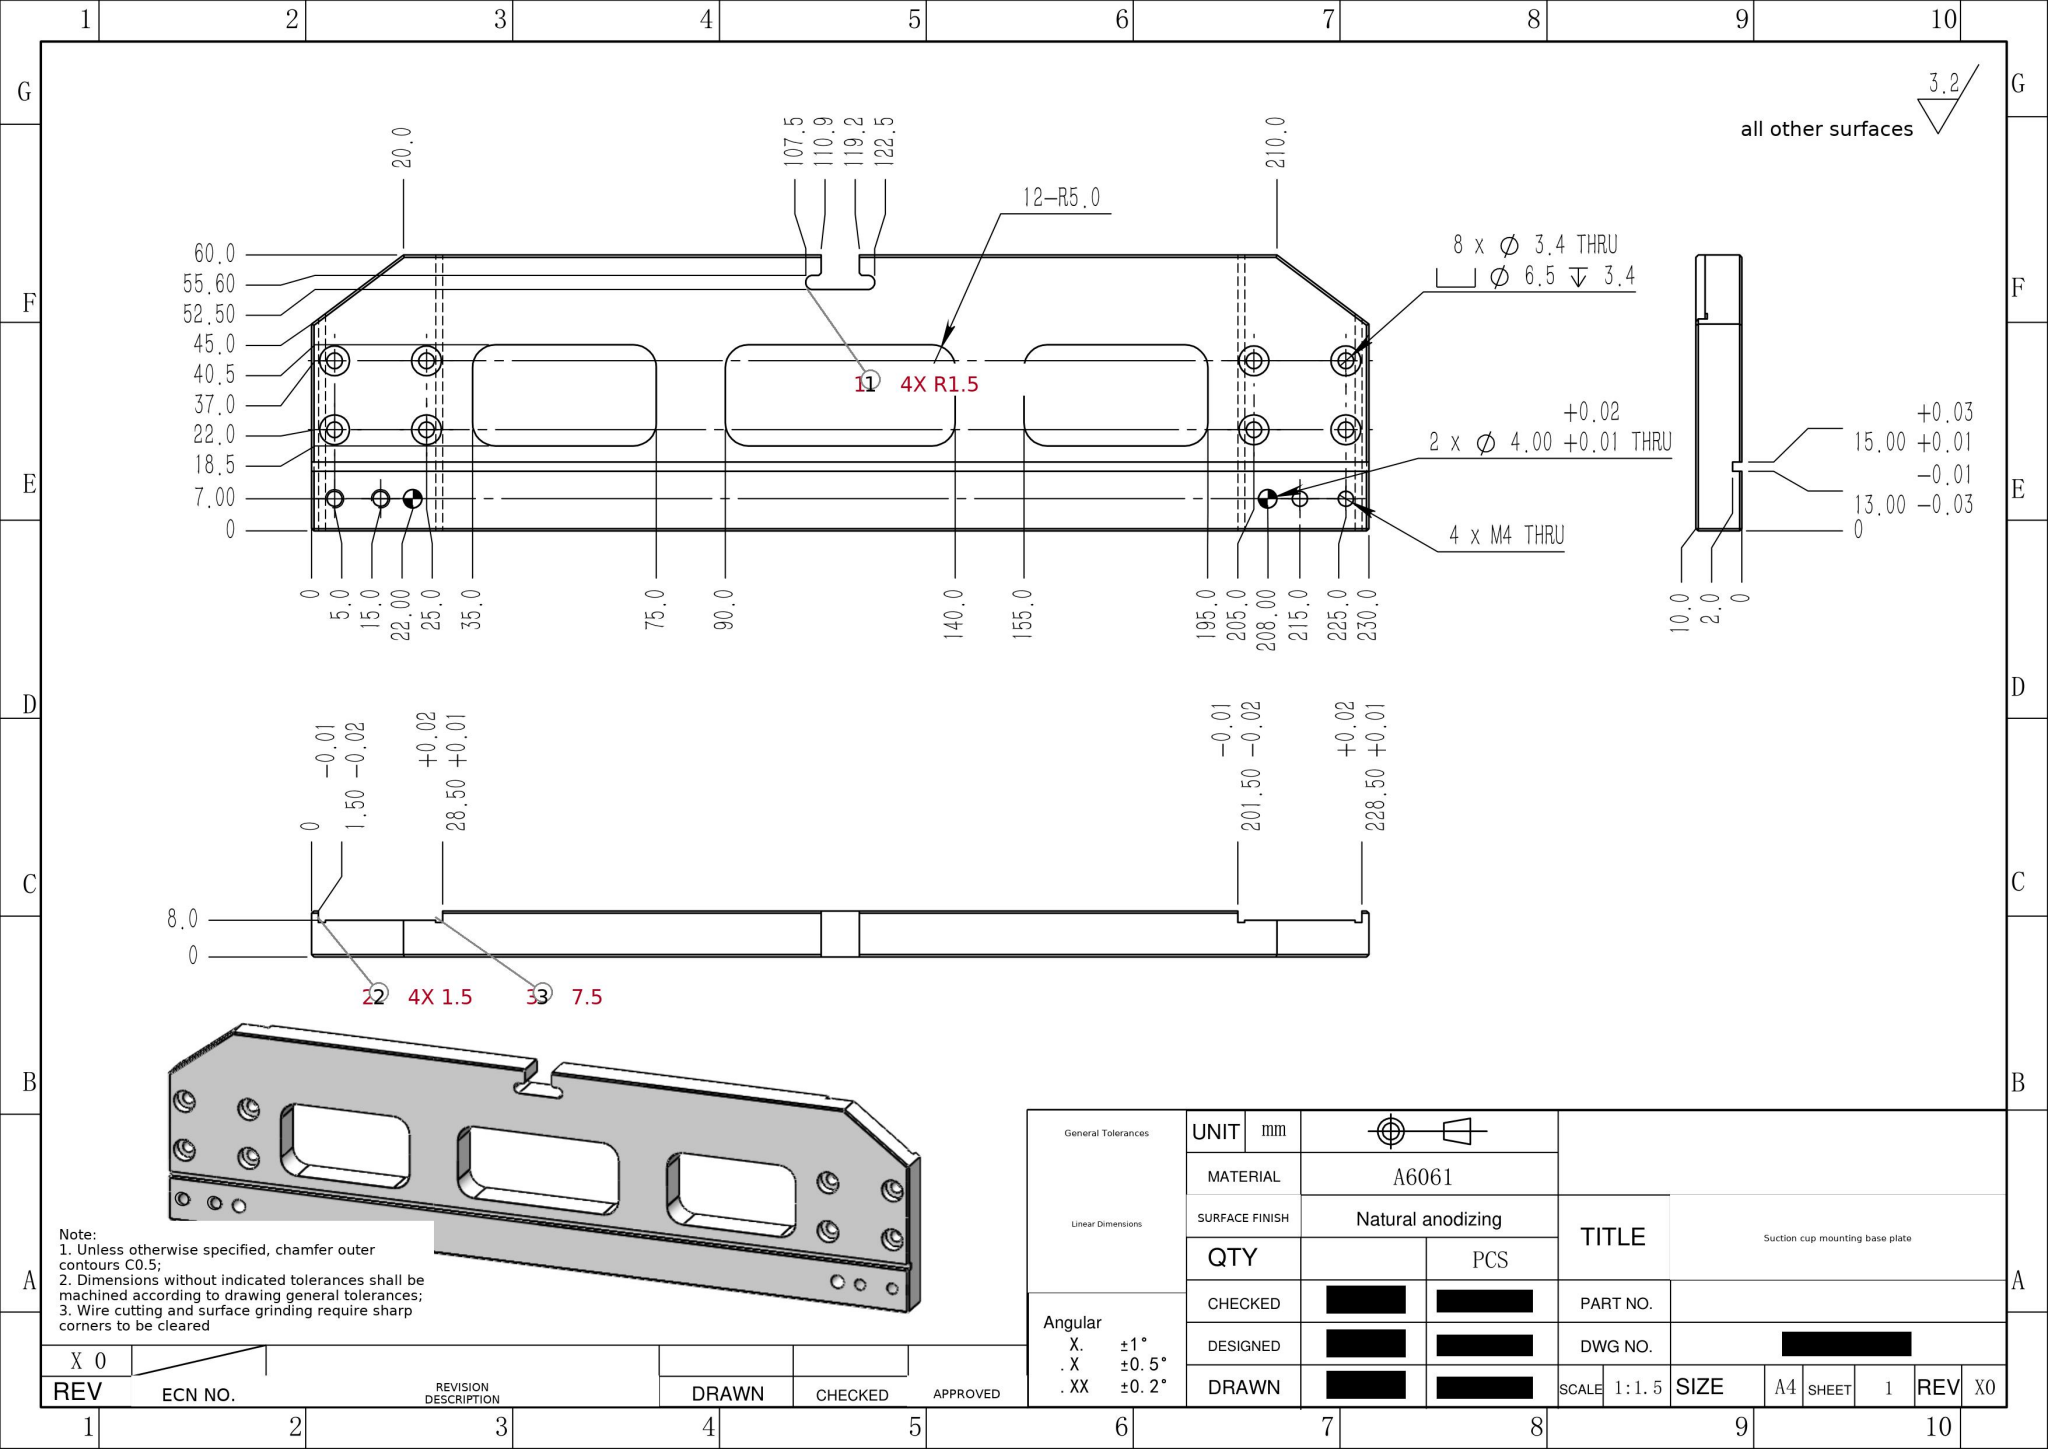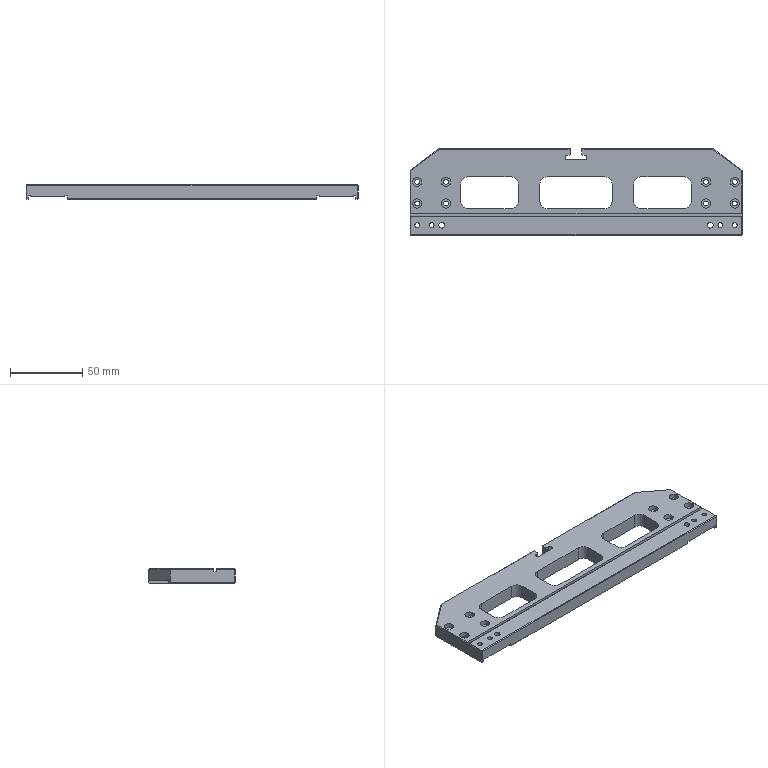Part | SolidWorks | mm | 1 solid | 142 faces | box 230 x 60 x 10 mm | volume 97348 mm3 | plane 82 | cylinder 60 | commonest cylinder face diameters 6.5 x16 3.4 x16 10 x12 3.3 x8 4 x4 3 x4
build123d program:
from build123d import *

# Parameters (mm, degrees)
SKETCH1_W                                       = 230
SKETCH1_H                                       = 60
BOSS_EXTRUDE1_DEPTH                             = 10
SKETCH2_W                                       = 27
SKETCH2_H                                       = 2
CUT_EXTRUDE1_DEPTH                              = 131.096
SKETCH3_W                                       = 1.5
SKETCH3_H                                       = 0.5
CUT_EXTRUDE2_DEPTH                              = 131.096
CUT_EXTRUDE3_DEPTH                              = 120.269
M3_HEX_SOCKET_HEAD_CAP_SCREW_CBORE1_D           = 3.4
M3_HEX_SOCKET_HEAD_CAP_SCREW_CBORE1_CBORE_D     = 6.5
M3_HEX_SOCKET_HEAD_CAP_SCREW_CBORE1_CBORE_DEPTH = 3.4
M4_TAPPED_HOLE1_D                               = 3.3
SKETCH10_W                                      = 2
SKETCH10_H                                      = 2
CUT_EXTRUDE5_DEPTH                              = 233.164
SKETCH11_W                                      = 40
SKETCH11_H                                      = 22
SKETCH11_W_2                                    = 50
CUT_EXTRUDE9_DEPTH                              = 120.269
CHAMFER1_SIZE                                   = 0.5
CUT_EXTRUDE10_DEPTH                             = 120.269
FILLET1_R                                       = 5
CHAMFER2_SIZE                                   = 0.5
FILLET2_R                                       = 1.5
SIZE_MM_DOWEL_PIN_HOLE1_D                       = 4


with BuildPart() as part:
    # Sketch1 → Boss-Extrude1 (new body)
    with BuildSketch(Plane.XY):
        Rectangle(SKETCH1_W, SKETCH1_H)
    extrude(amount=-BOSS_EXTRUDE1_DEPTH)

    # Sketch2 → Cut-Extrude1 (cut, through all)
    with BuildSketch(Plane(origin=(0, 30, 0), x_dir=(1, 0, 0), z_dir=(0, 1, 0))):
        with Locations((-100, 9)):
            Rectangle(SKETCH2_W, SKETCH2_H)
        with Locations((100, 9)):
            Rectangle(SKETCH2_W, SKETCH2_H)
    extrude(amount=-CUT_EXTRUDE1_DEPTH, mode=Mode.SUBTRACT)

    # Sketch3 → Cut-Extrude2 (cut, through all)
    with BuildSketch(Plane(origin=(0, 30, 0), x_dir=(1, 0, 0), z_dir=(0, 1, 0))):
        with Locations((-87.25, 7.75)):
            Rectangle(SKETCH3_W, SKETCH3_H)
        with Locations((-112.75, 7.75)):
            Rectangle(SKETCH3_W, SKETCH3_H)
        with Locations((87.25, 7.75)):
            Rectangle(SKETCH3_W, SKETCH3_H)
        with Locations((112.75, 7.75)):
            Rectangle(SKETCH3_W, SKETCH3_H)
    extrude(amount=-CUT_EXTRUDE2_DEPTH, mode=Mode.SUBTRACT)

    # Sketch4 → Cut-Extrude3 (cut, through all)
    with BuildSketch(Plane.XY):
        Polygon((-115, 30), (-95, 30), (-115, 15), align=None)
        Polygon((115, 15), (115, 30), (95, 30), align=None)
    extrude(amount=-CUT_EXTRUDE3_DEPTH, mode=Mode.SUBTRACT)

    # M3 Hex Socket Head Cap Screw CBORE1 (through all)
    with Locations(Plane.XY):
        with Locations((-110, 7), (-90, 7), (-90, -8), (-110, -8), (110, -8), (90, -8), (90, 7), (110, 7)):
            CounterBoreHole(M3_HEX_SOCKET_HEAD_CAP_SCREW_CBORE1_D / 2, M3_HEX_SOCKET_HEAD_CAP_SCREW_CBORE1_CBORE_D / 2, M3_HEX_SOCKET_HEAD_CAP_SCREW_CBORE1_CBORE_DEPTH)

    # M4 Tapped Hole1 (through all)
    with Locations(Plane.XY):
        with Locations((-100, -23), (-110, -23), (110, -23), (100, -23)):
            Hole(M4_TAPPED_HOLE1_D / 2)

    # Sketch10 → Cut-Extrude5 (cut, through all)
    with BuildSketch(Plane(origin=(115, 0, 0), x_dir=(0, 0, -1), z_dir=(1, 0, 0))):
        with Locations((1, -16)):
            Rectangle(SKETCH10_W, SKETCH10_H)
    extrude(amount=-CUT_EXTRUDE5_DEPTH, mode=Mode.SUBTRACT)

    # Sketch11 → Cut-Extrude9 (cut, through all)
    with BuildSketch(Plane.XY):
        with Locations((60, -0.5)):
            Rectangle(SKETCH11_W, SKETCH11_H)
        with Locations((0, -0.5)):
            Rectangle(SKETCH11_W_2, SKETCH11_H)
        with Locations((-60, -0.5)):
            Rectangle(SKETCH11_W, SKETCH11_H)
    extrude(amount=-CUT_EXTRUDE9_DEPTH, mode=Mode.SUBTRACT)

    # Chamfer1
    chamfer1_edges = [part.edges().sort_by_distance(p)[0] for p in [
        (-115, 0, 0),
        (-115, -7.5, -10),
        (-114.25, 15.562, -10),
        (-105, 22.5, 0),
        (0, 30, 0),
        (114.25, 15.562, -10),
        (105, 22.5, 0),
        (-114.25, -30, -10),
        (0, -30, -10),
        (-115, -23.5, 0),
        (115, 0, 0),
        (114.25, -30, -10),
        (0, 30, -10),
        (115, -7.5, -10),
        (0, -30, 0),
        (115, -23.5, 0),
        (115, -30, -5),
        (-115, -30, -5),
    ]]
    chamfer(chamfer1_edges, length=CHAMFER1_SIZE)

    # Sketch12 → Cut-Extrude10 (cut, through all)
    with BuildSketch(Plane.XY):
        Polygon((-4.15, 30), (4.15, 30), (4.15, 25.6), (7.5, 25.6), (7.5, 22.5), (-7.5, 22.5), (-7.5, 25.6), (-4.15, 25.6), align=None)
    extrude(amount=-CUT_EXTRUDE10_DEPTH, mode=Mode.SUBTRACT)

    # Fillet1
    fillet1_edges = [part.edges().sort_by_distance(p)[0] for p in [
        (-25, -11.5, -5),
        (-25, 10.5, -5),
        (25, 10.5, -5),
        (25, -11.5, -5),
        (-80, -11.5, -5),
        (-80, 10.5, -5),
        (-40, 10.5, -5),
        (-40, -11.5, -5),
        (40, 10.5, -5),
        (80, 10.5, -5),
        (80, -11.5, -5),
        (40, -11.5, -5),
    ]]
    fillet(fillet1_edges, radius=FILLET1_R)

    # Chamfer2
    chamfer2_edges = [part.edges().sort_by_distance(p)[0] for p in [
        (4.15, 25.6, -5),
        (-4.15, 25.6, -5),
    ]]
    chamfer(chamfer2_edges, length=CHAMFER2_SIZE)

    # Fillet2
    fillet2_edges = [part.edges().sort_by_distance(p)[0] for p in [
        (7.5, 25.6, -5),
        (7.5, 22.5, -5),
        (-7.5, 22.5, -5),
        (-7.5, 25.6, -5),
    ]]
    fillet(fillet2_edges, radius=FILLET2_R)

    # Size mm Dowel Pin Hole1 (through all)
    with Locations(Plane.XY):
        with Locations((-93, -23), (93, -23)):
            Hole(SIZE_MM_DOWEL_PIN_HOLE1_D / 2)


solid = part.part